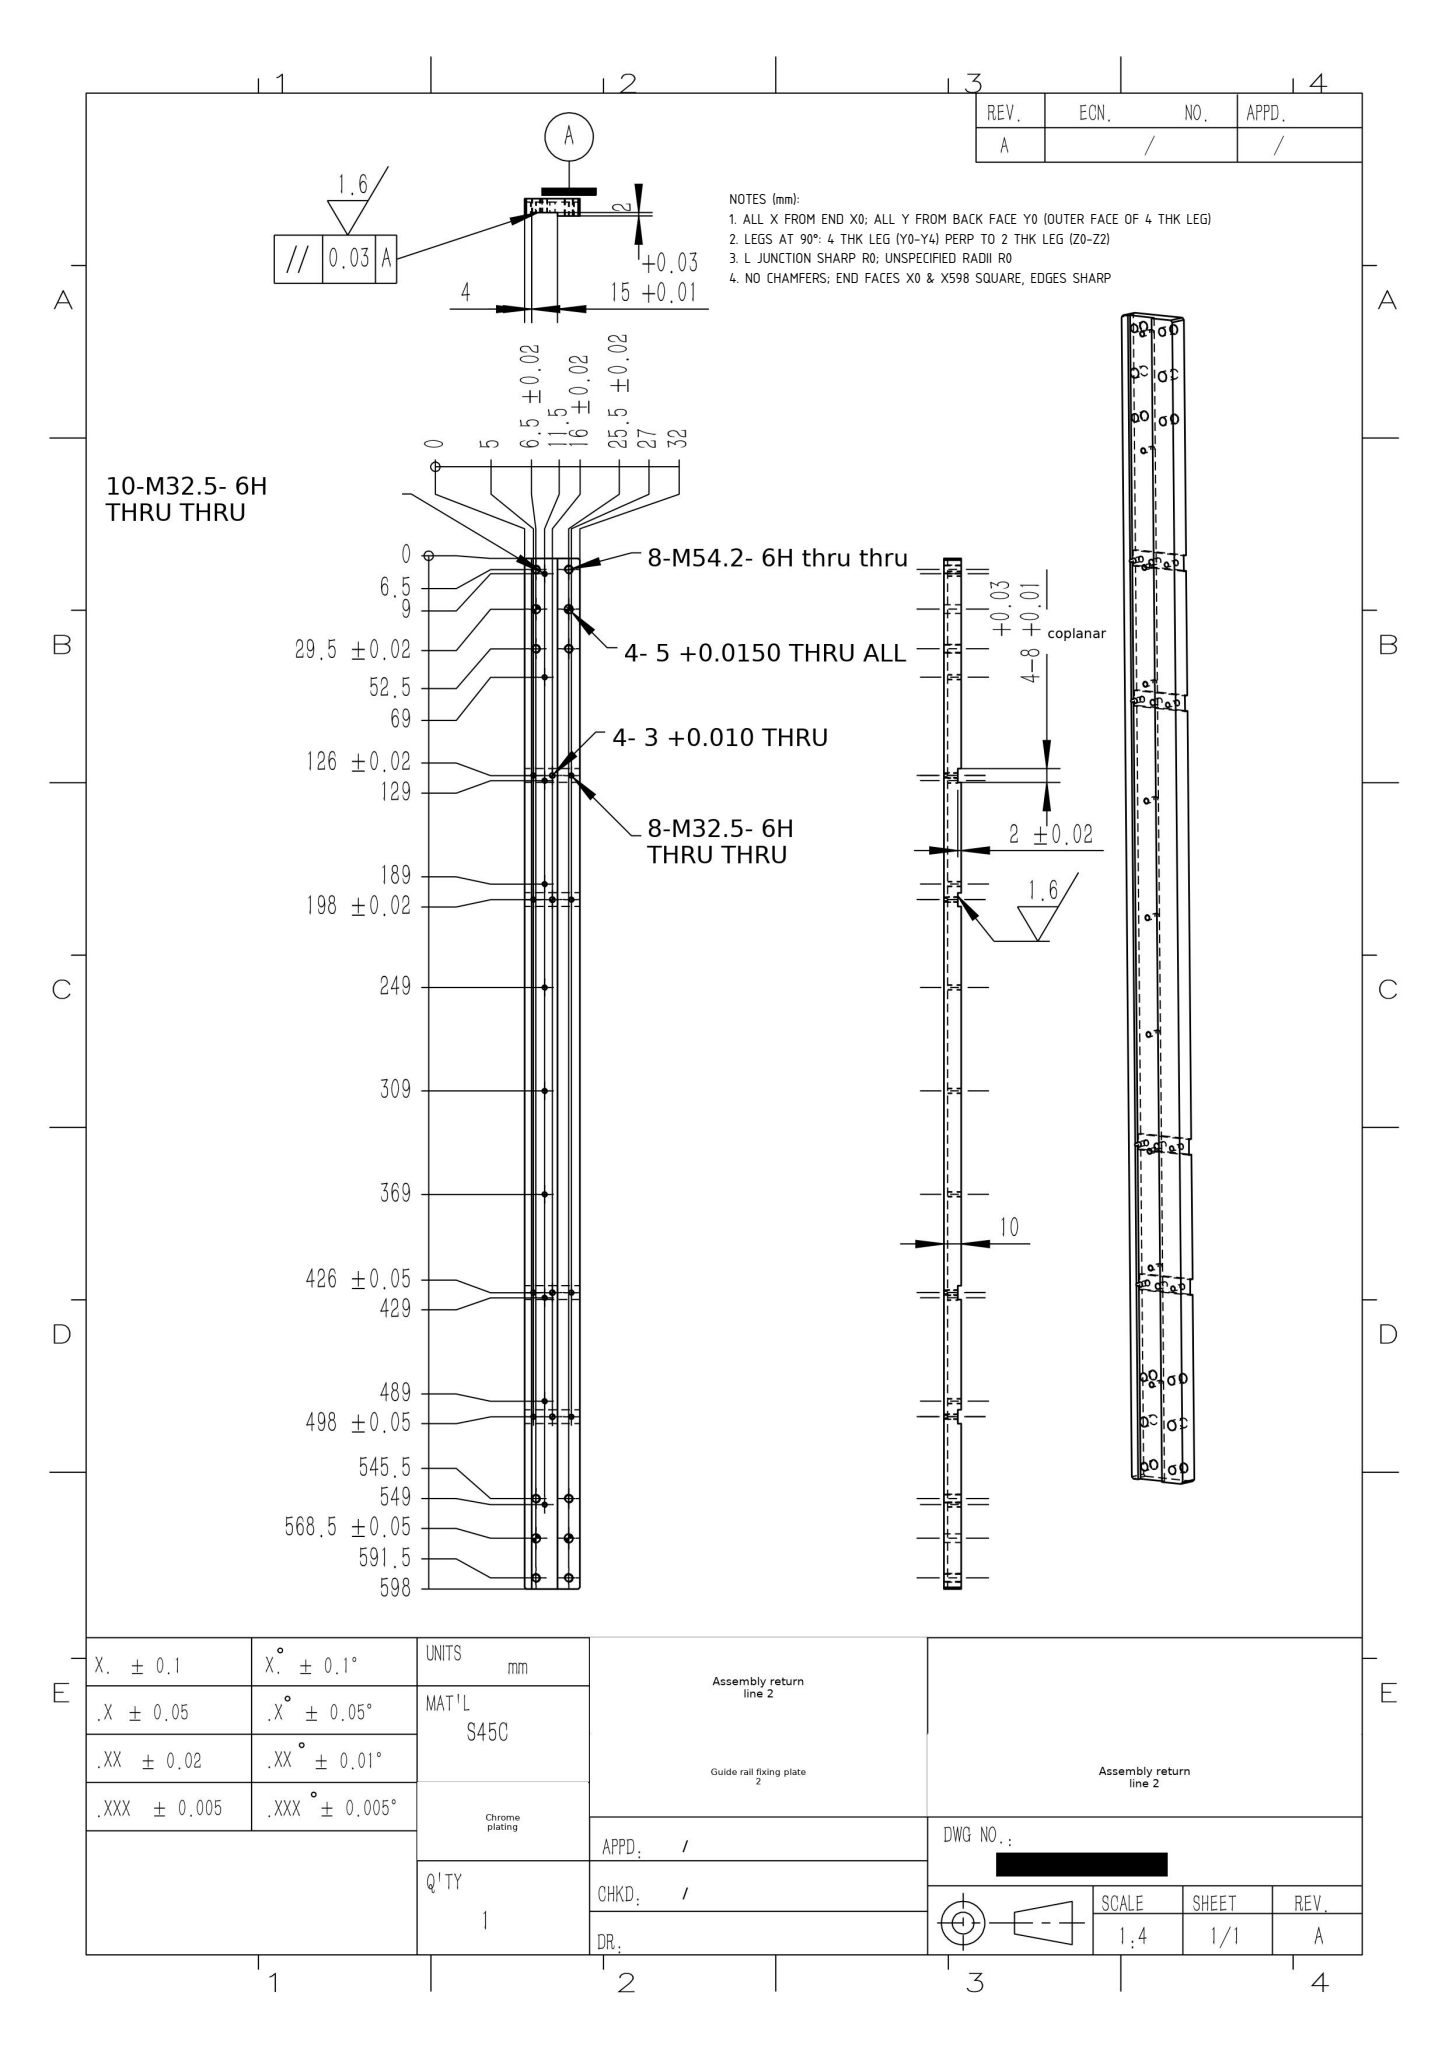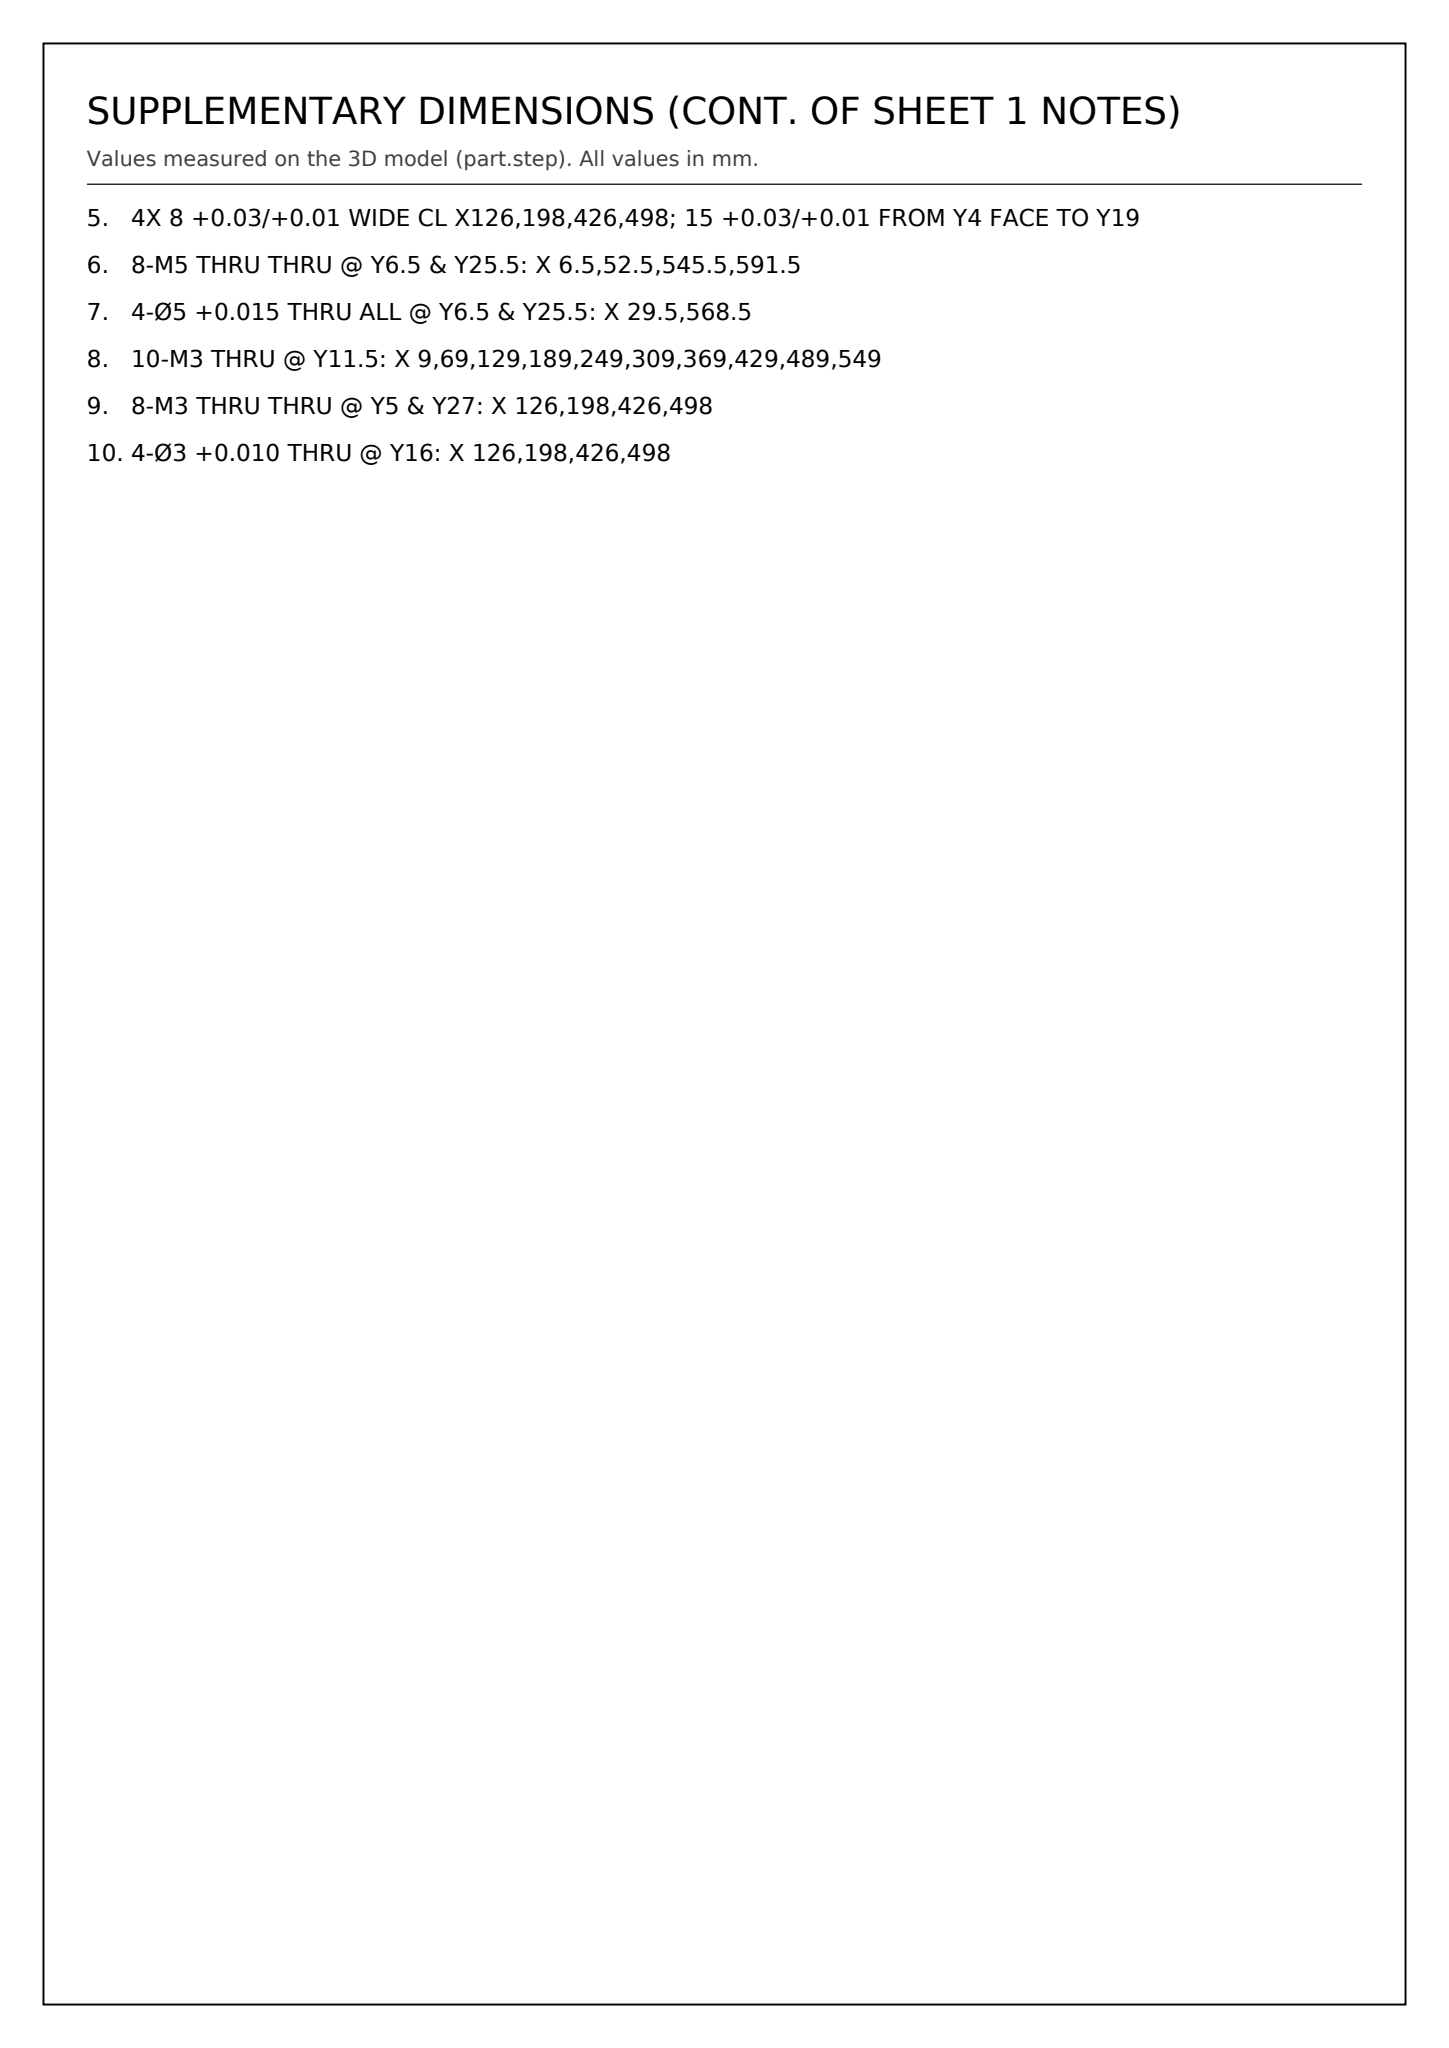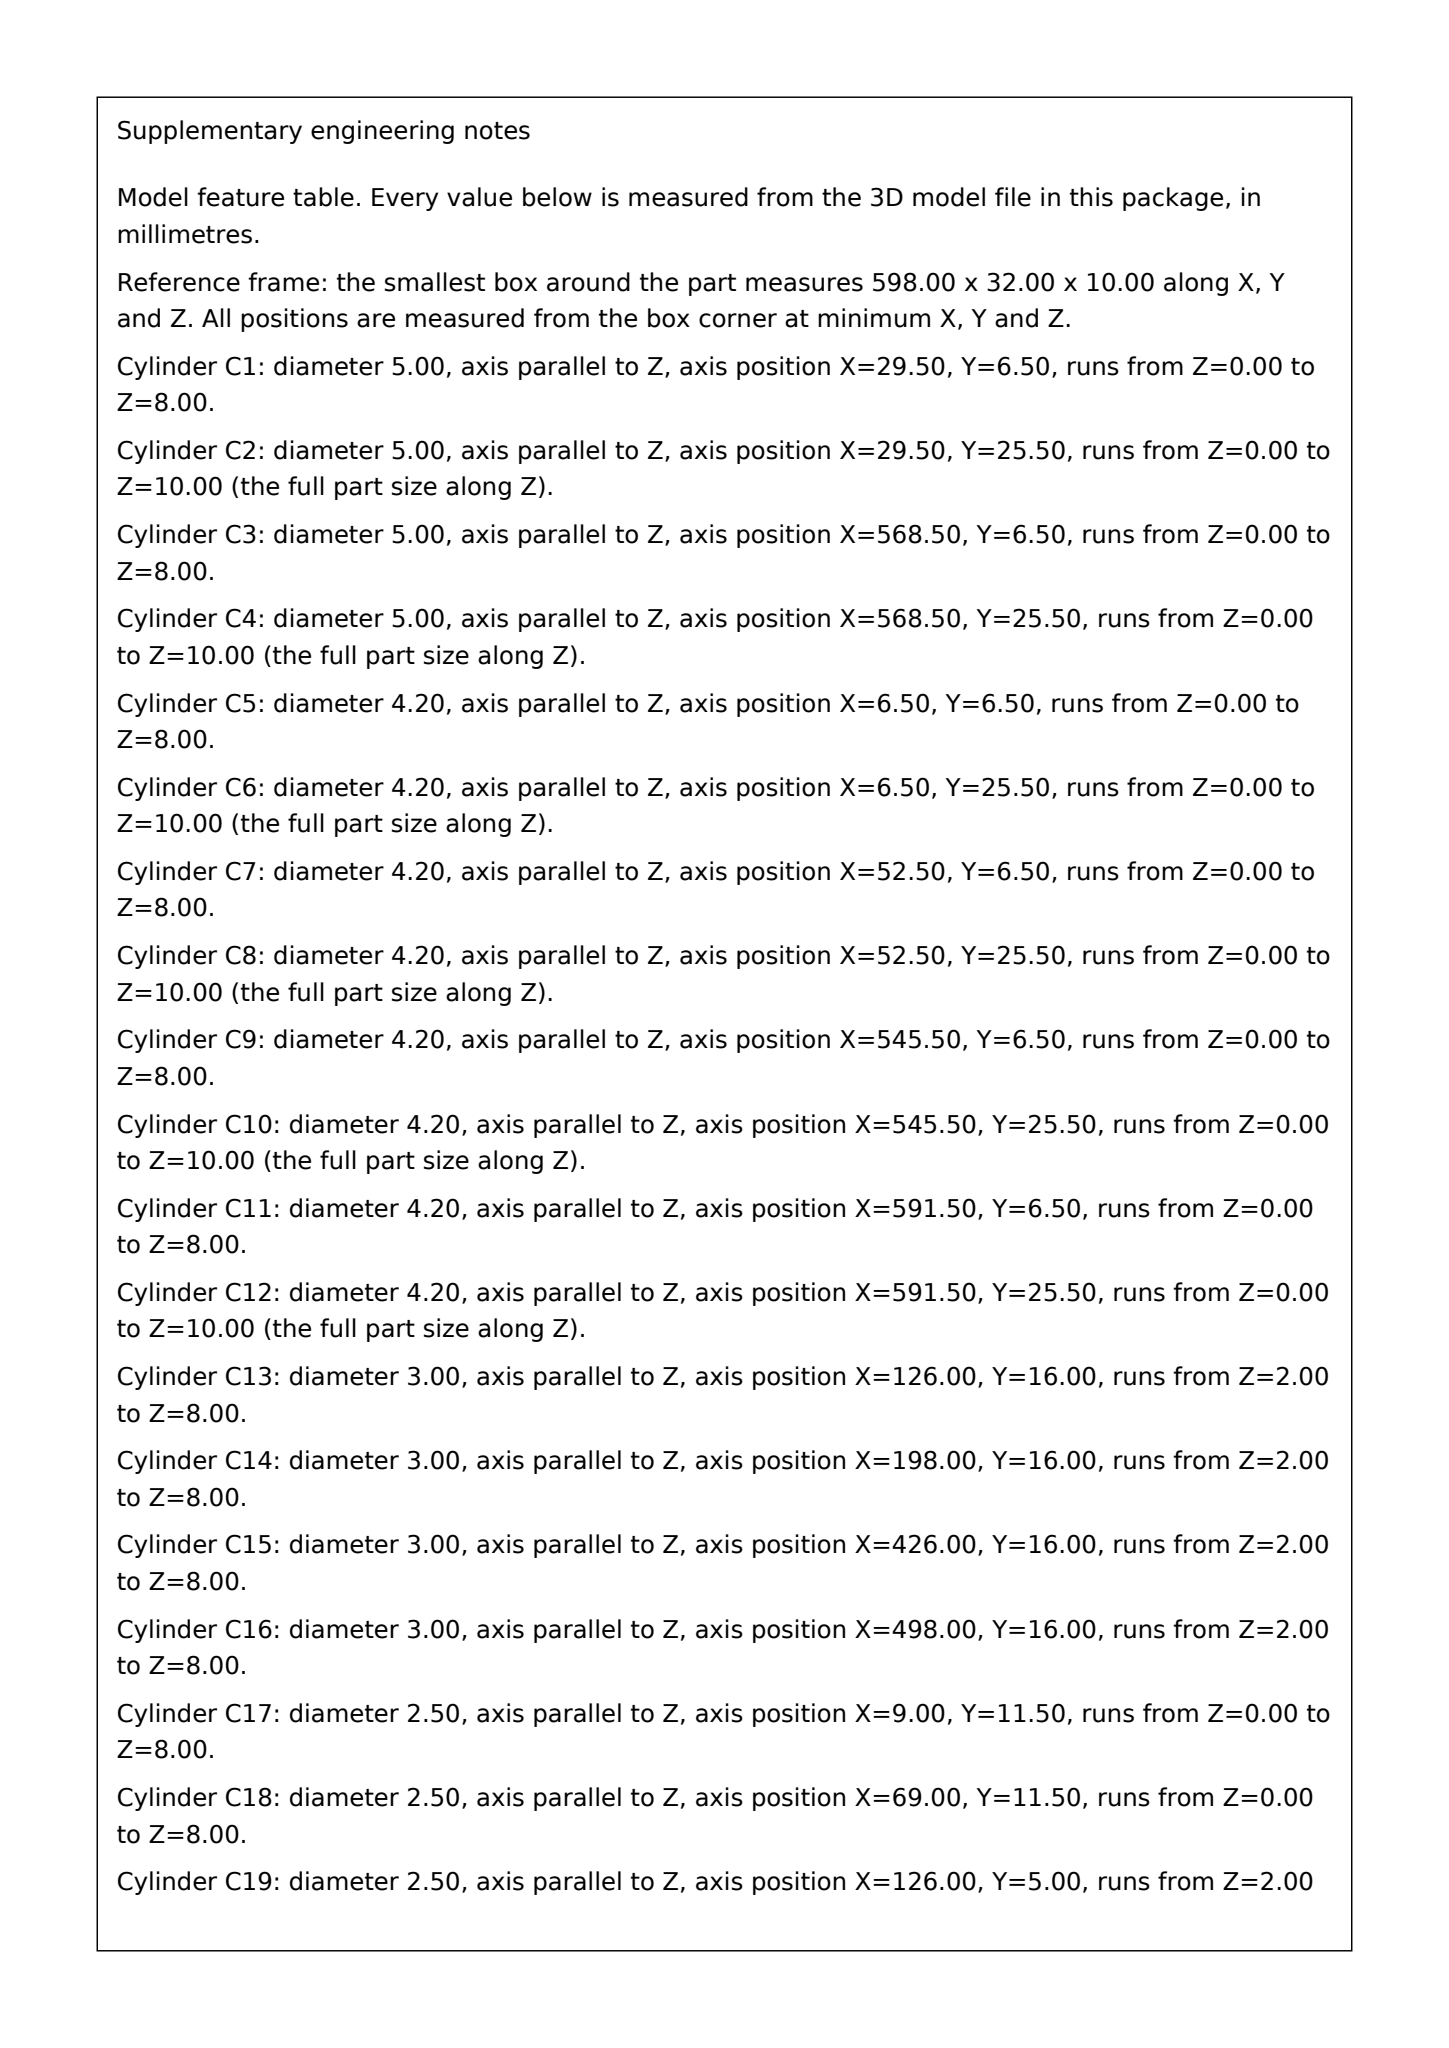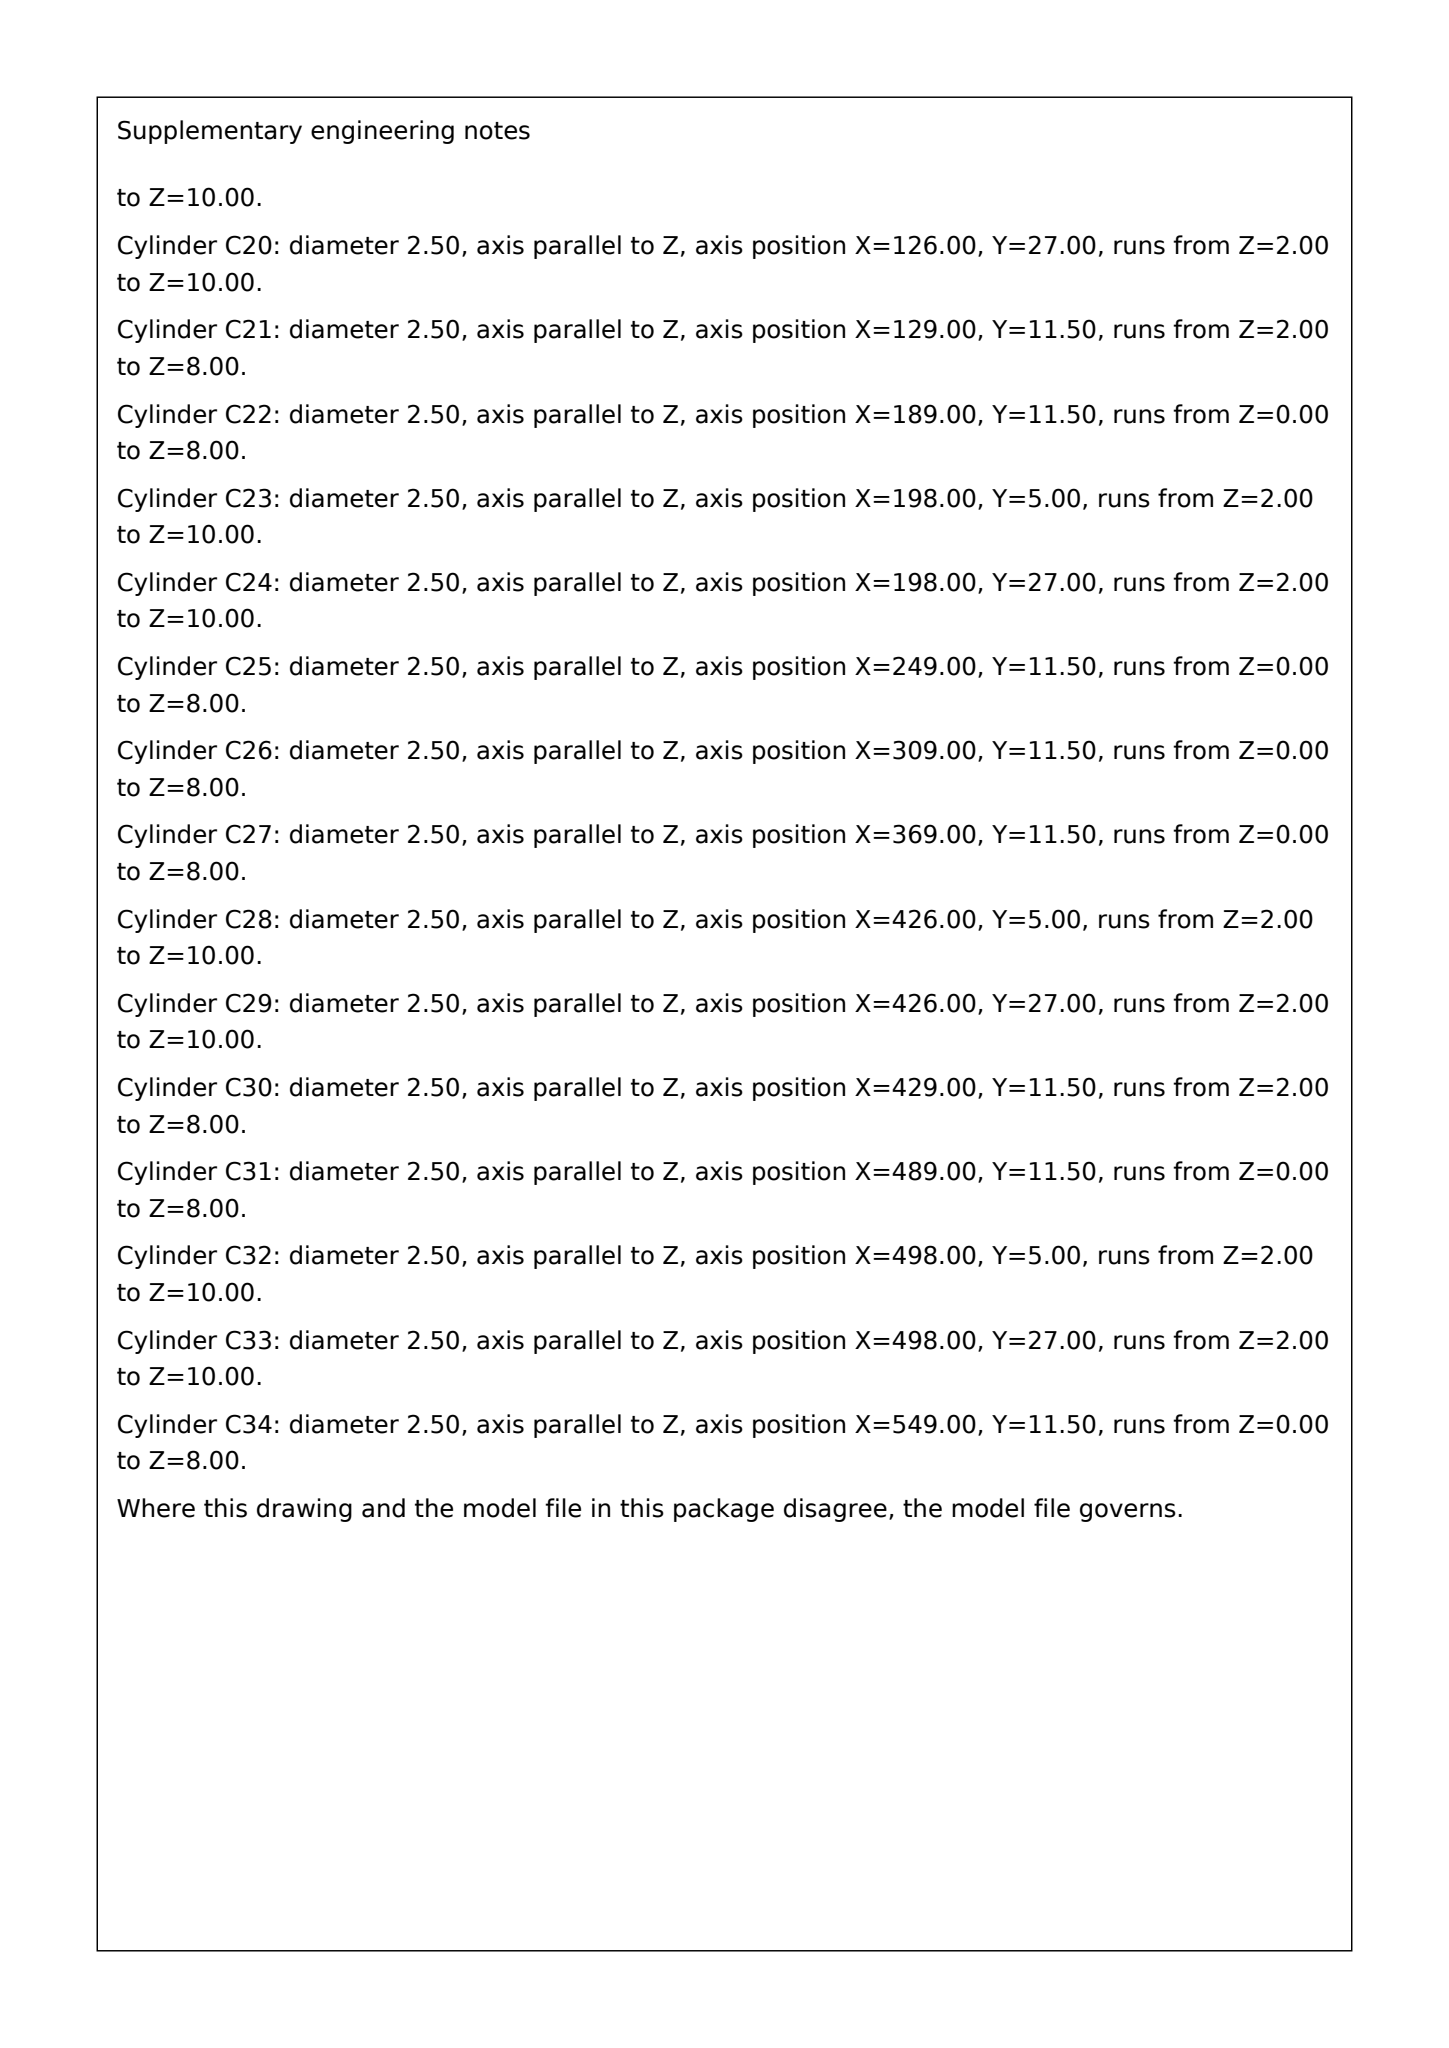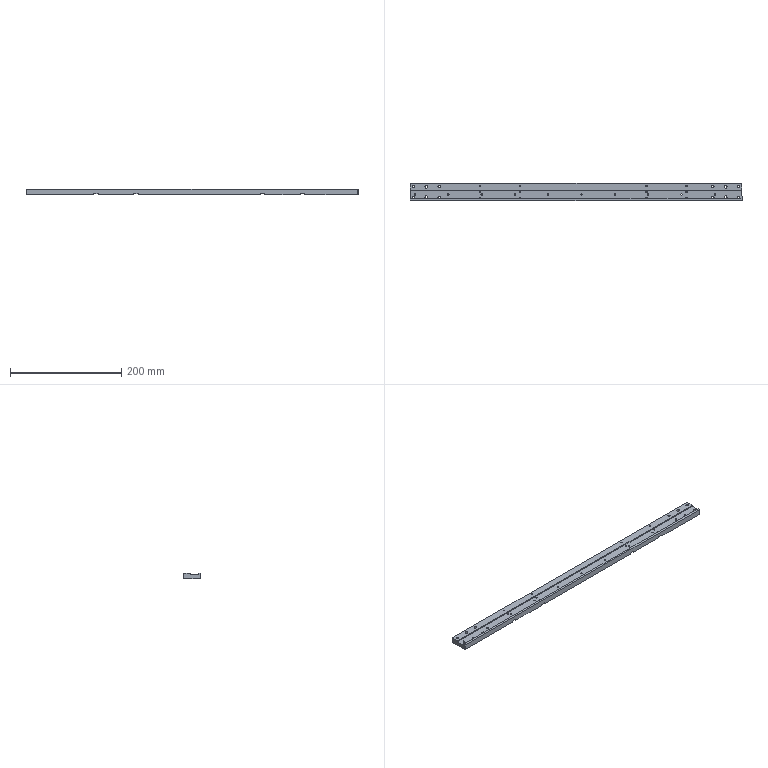Part | SolidWorks | mm | 1 solid | 104 faces | box 598 x 32 x 10 mm | volume 168828 mm3 | cylinder 68 | plane 36 | commonest cylinder face diameters 2.5 x36 4.2 x16 5 x8 3 x8
Drawing notes:
ALL X FROM END X0; ALL Y FROM BACK FACE Y0 (OUTER FACE OF 4 THK LEG) | from the solid: bbox min corner = x0 end face, y0 outer face of 4 thk leg
LEGS AT 90°: 4 THK LEG (Y0-Y4) PERP TO 2 THK LEG (Z0-Z2) | from the solid: axis_planes normals x/y/z only: y=0,4 and z=0,2 mutually orthogonal
L JUNCTION SHARP R0; UNSPECIFIED RADII R0 | from the solid: fillet_radii: [] (empty) - no filleted edges in model
NO CHAMFERS; END FACES X0 & X598 SQUARE, EDGES SHARP | from the solid: cones: [] (none); planes x=0 and x=598 normal to axis
4X 8 +0.03/+0.01 WIDE CL X126,198,426,498; 15 +0.03/+0.01 FROM Y4 FACE TO Y19 | from the solid: x planes 122/130,194/202,422/430,494/502 -> 8 wide; y=4 and coplanar y=19, 19-4=15
8-M5 THRU THRU @ Y6.5 & Y25.5: X 6.5,52.5,545.5,591.5 | from the solid: Ø4.2 (M5 tap drill) holes at y=6.5/25.5, x=6.5,52.5,545.5,591.5
4-Ø5 +0.015 THRU ALL @ Y6.5 & Y25.5: X 29.5,568.5 | from the solid: Ø5.0 holes at y=6.5/25.5, x=29.5 and 568.5
10-M3 THRU @ Y11.5: X 9,69,129,189,249,309,369,429,489,549 | from the solid: Ø2.5 holes at y=11.5, x=9,69,129,189,249,309,369,429,489,549
8-M3 THRU THRU @ Y5 & Y27: X 126,198,426,498 | from the solid: Ø2.5 holes at y=5 and y=27, x=126,198,426,498
4-Ø3 +0.010 THRU @ Y16: X 126,198,426,498 | from the solid: Ø3.0 holes at y=16, x=126,198,426,498